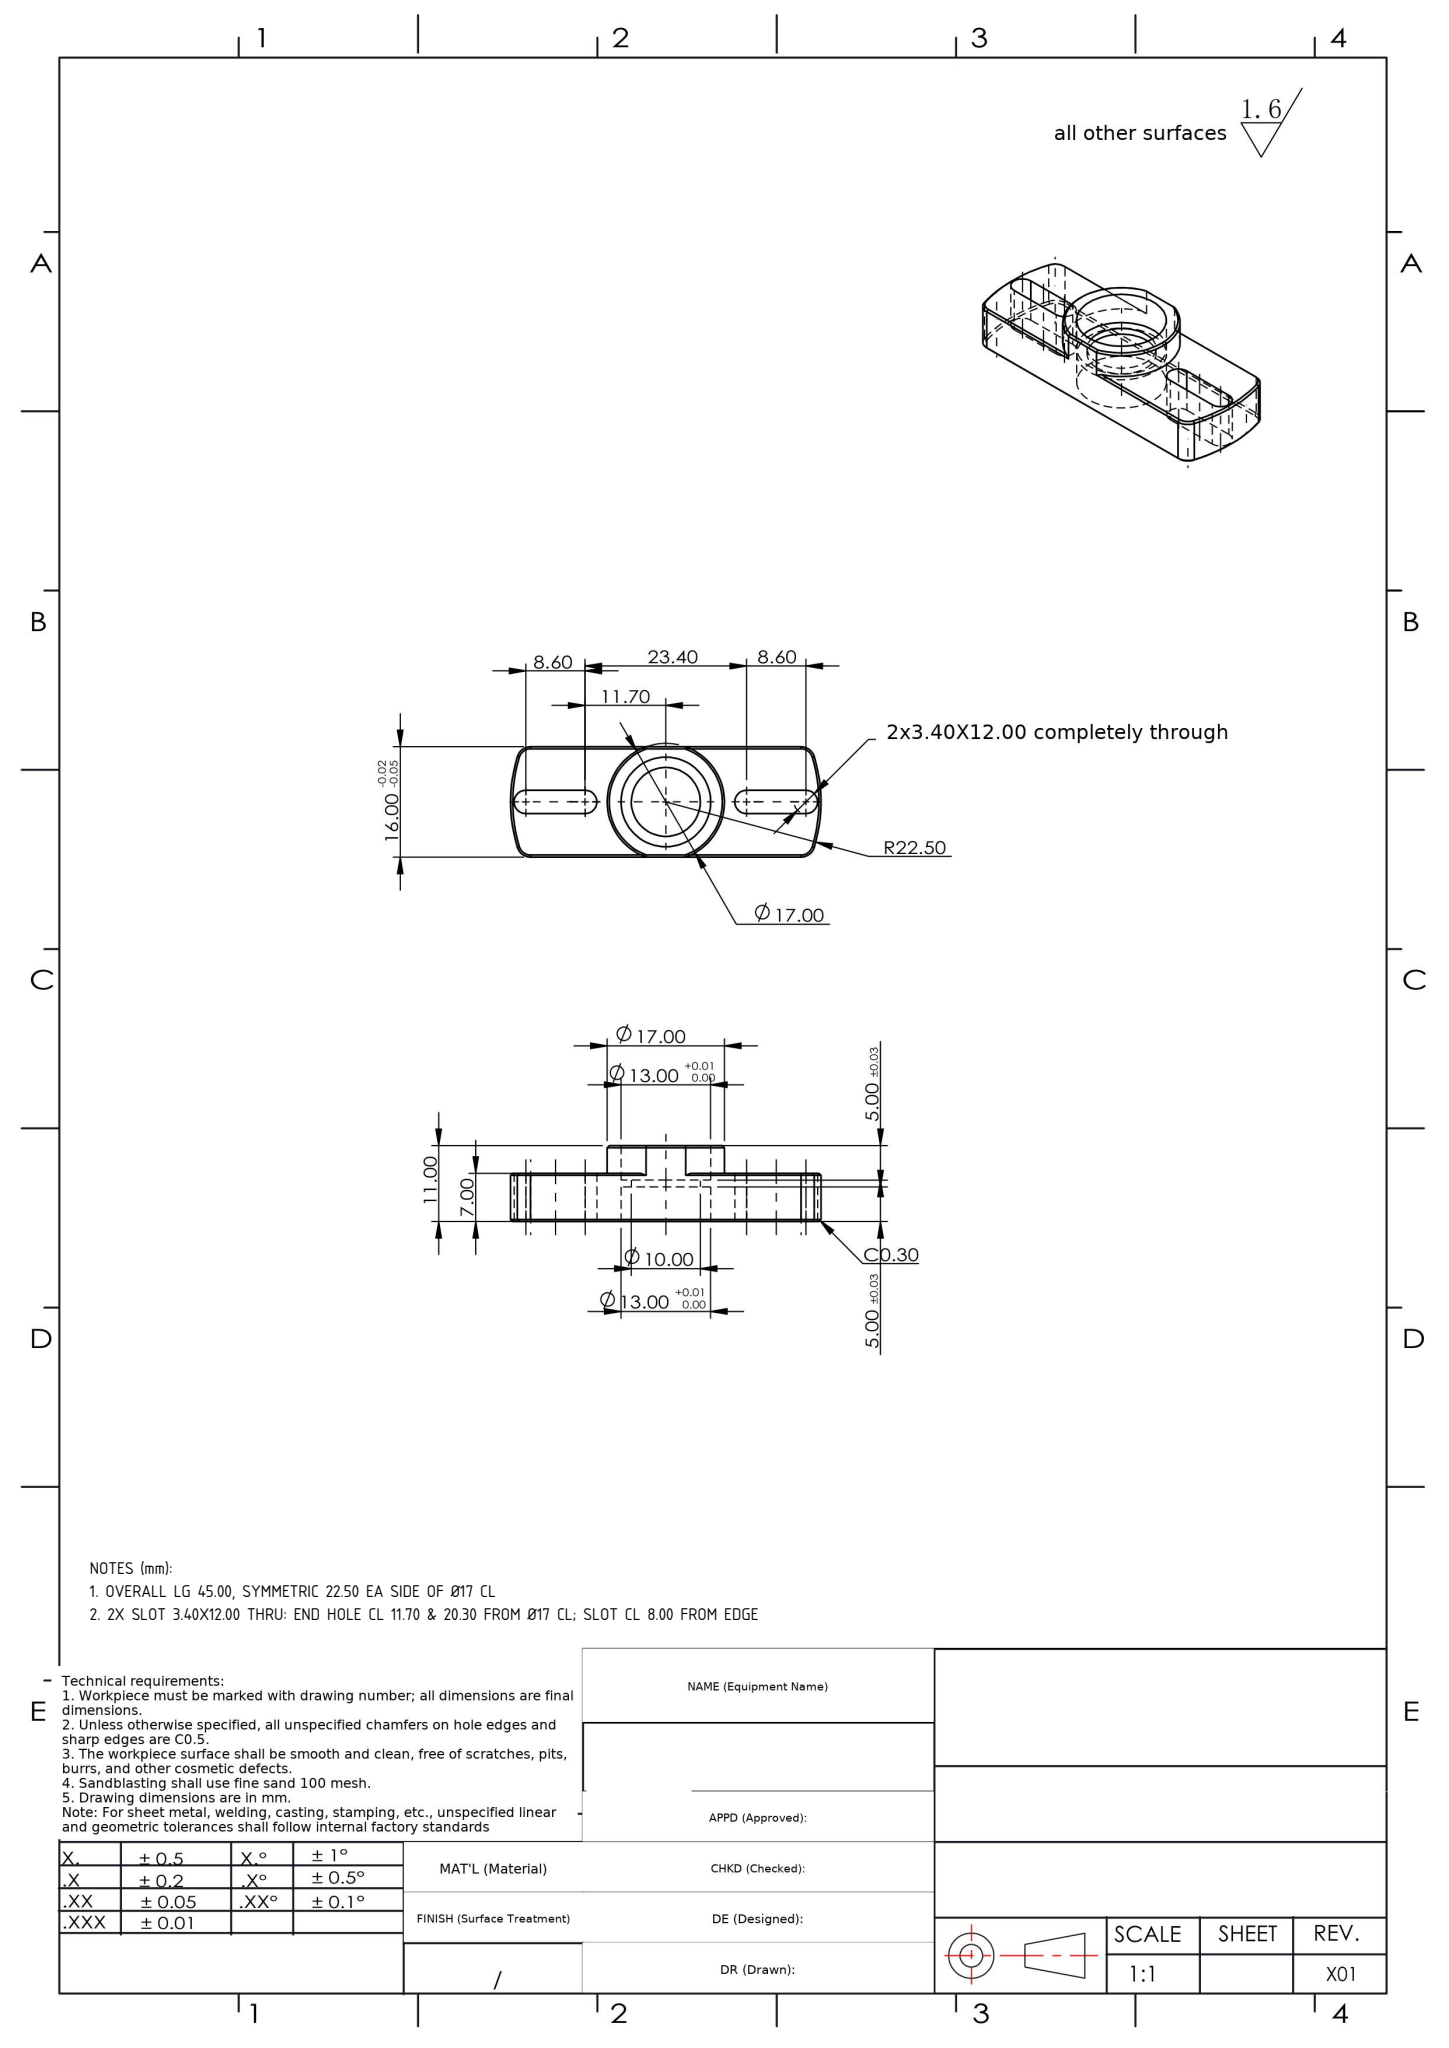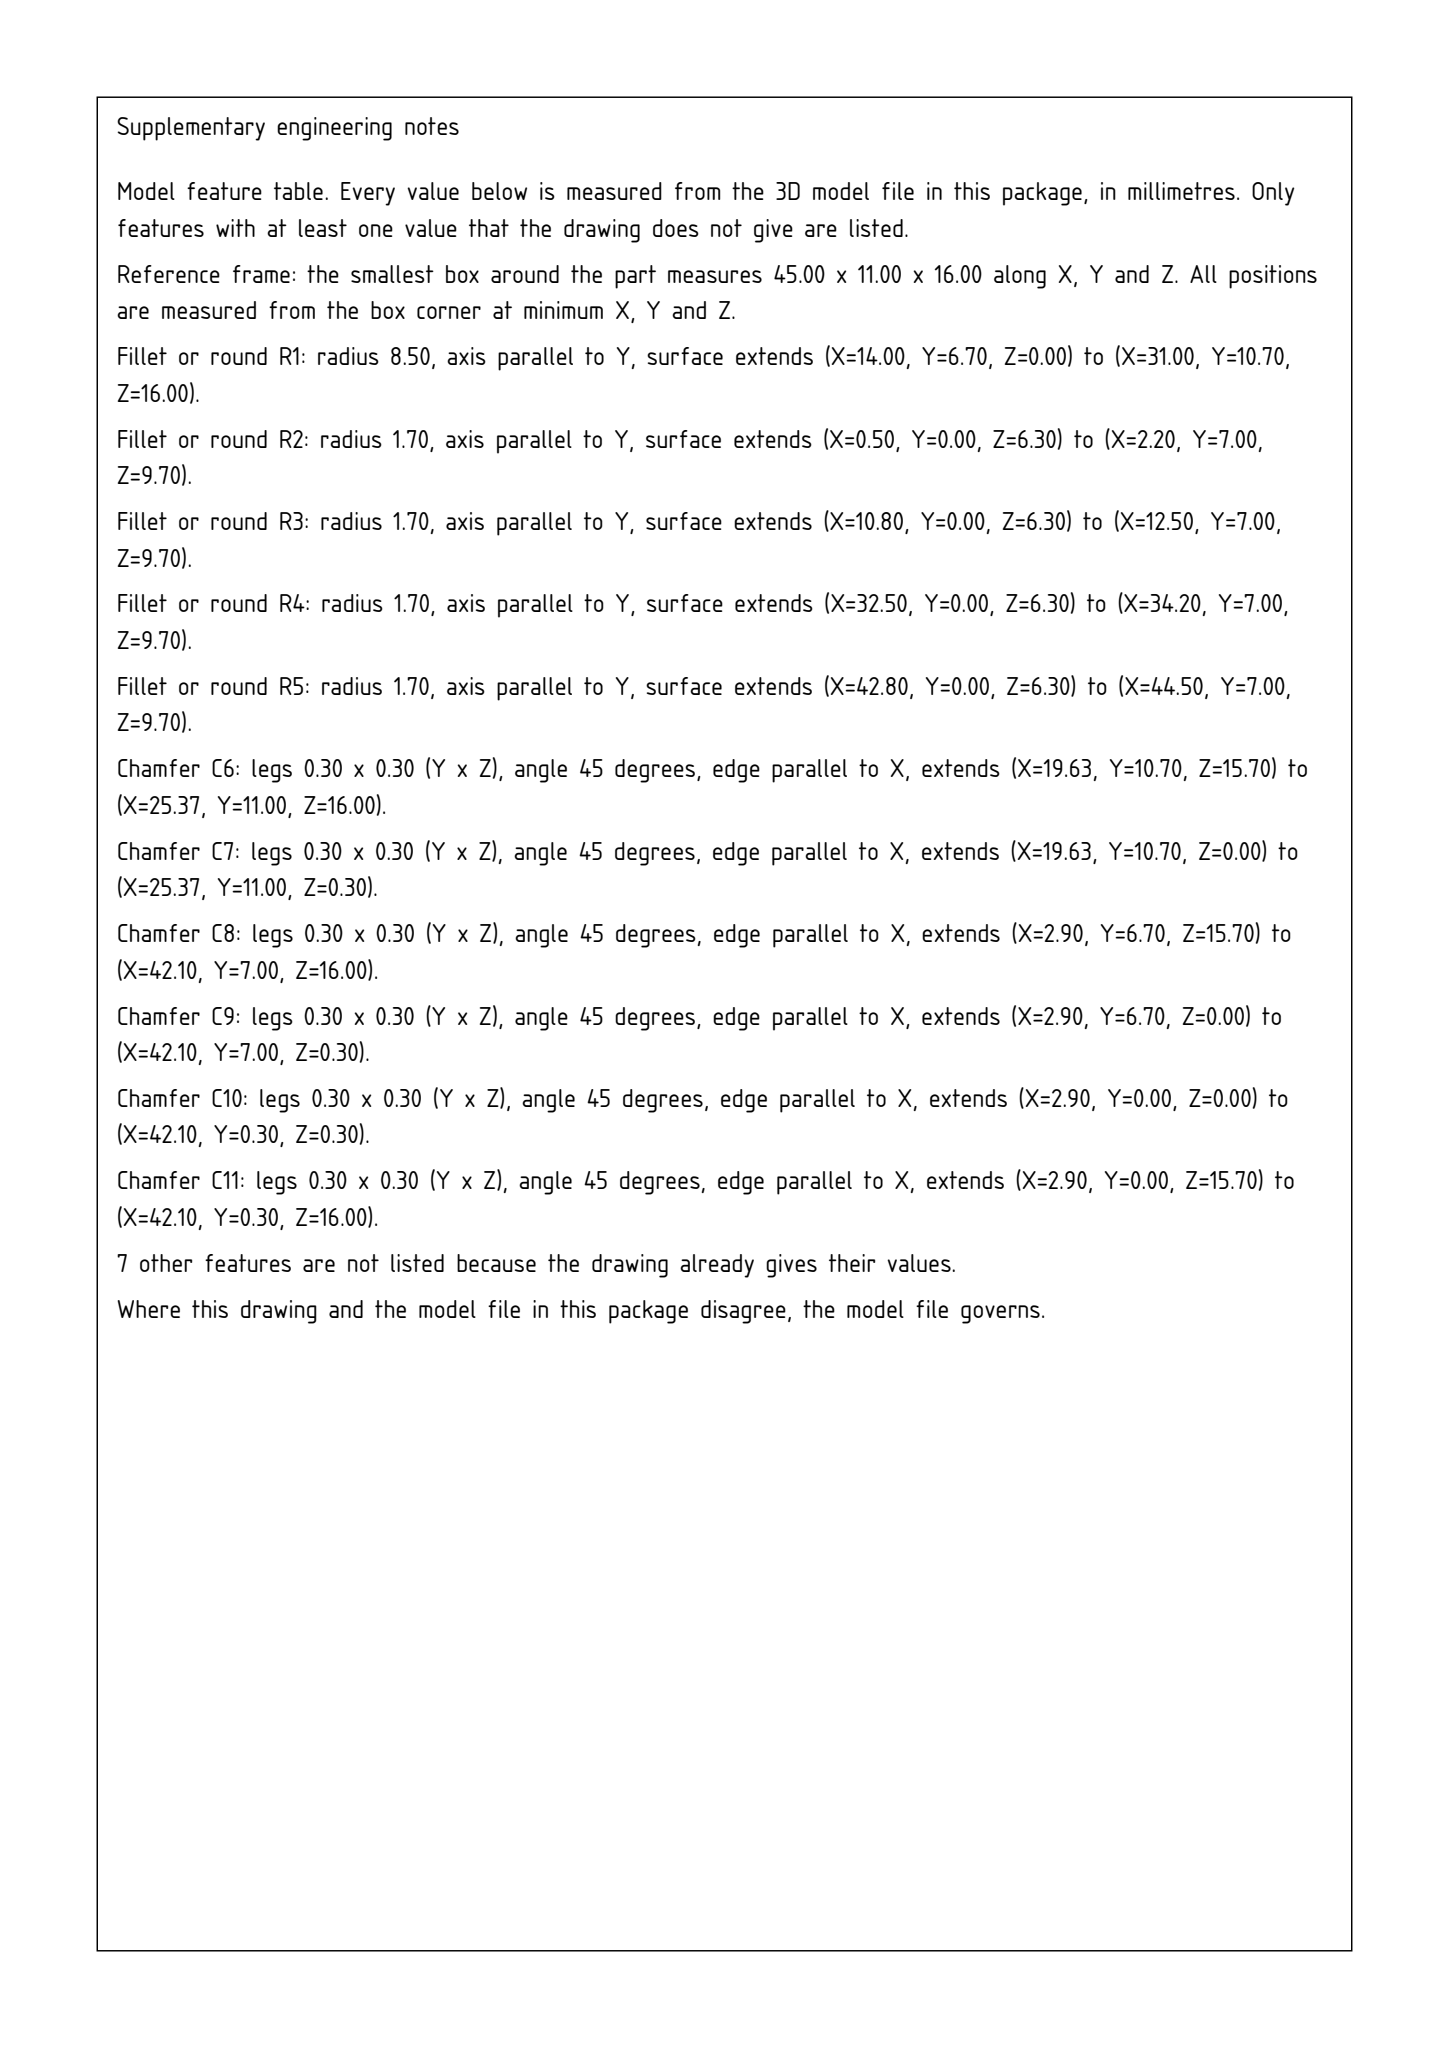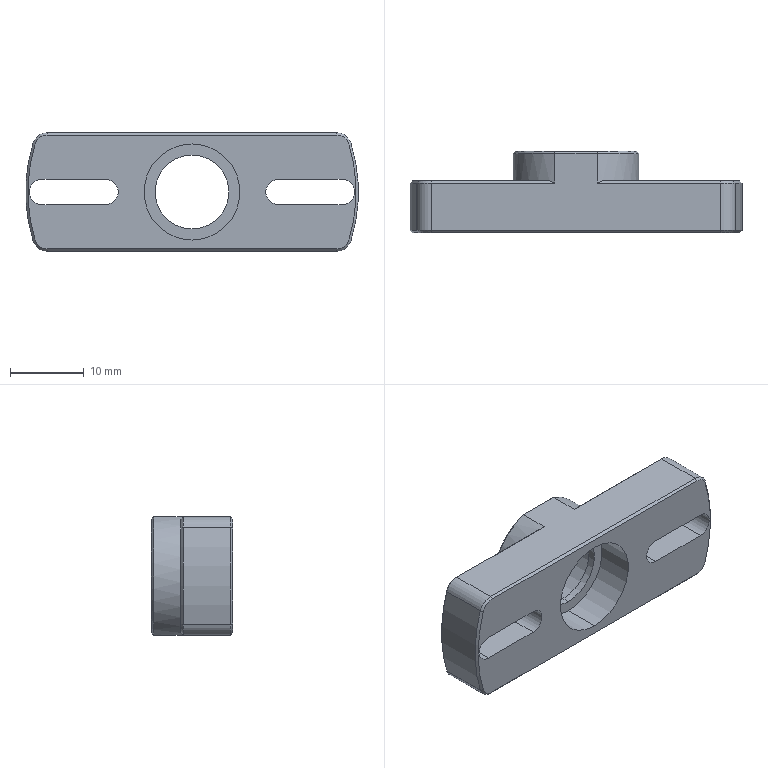Part | SolidWorks | mm | 1 solid | 52 faces | box 45 x 11 x 16 mm | volume 3859 mm3 | plane 20 | cylinder 18 | cone 14 | commonest cylinder face diameters 13 x4 3.4 x4 4 x4 10 x2 17 x2 45 x2
Drawing notes:
OVERALL LG 45.00, SYMMETRIC 22.50 EA SIDE OF Ø17 CL | from the solid: bbox_xyz x=45.0; Ø17/Ø13 bore axis at x=22.5, R22.50 end arcs tangent
2X SLOT 3.40X12.00 THRU: END HOLE CL 11.70 & 20.30 FROM Ø17 CL; SLOT CL 8.00 FROM EDGE | from the solid: Ø3.4 holes at x=2.2,10.8,34.2,42.8 vs Ø17 CL x=22.5 -> 11.70/20.30; z=8.0 of 16.0 width